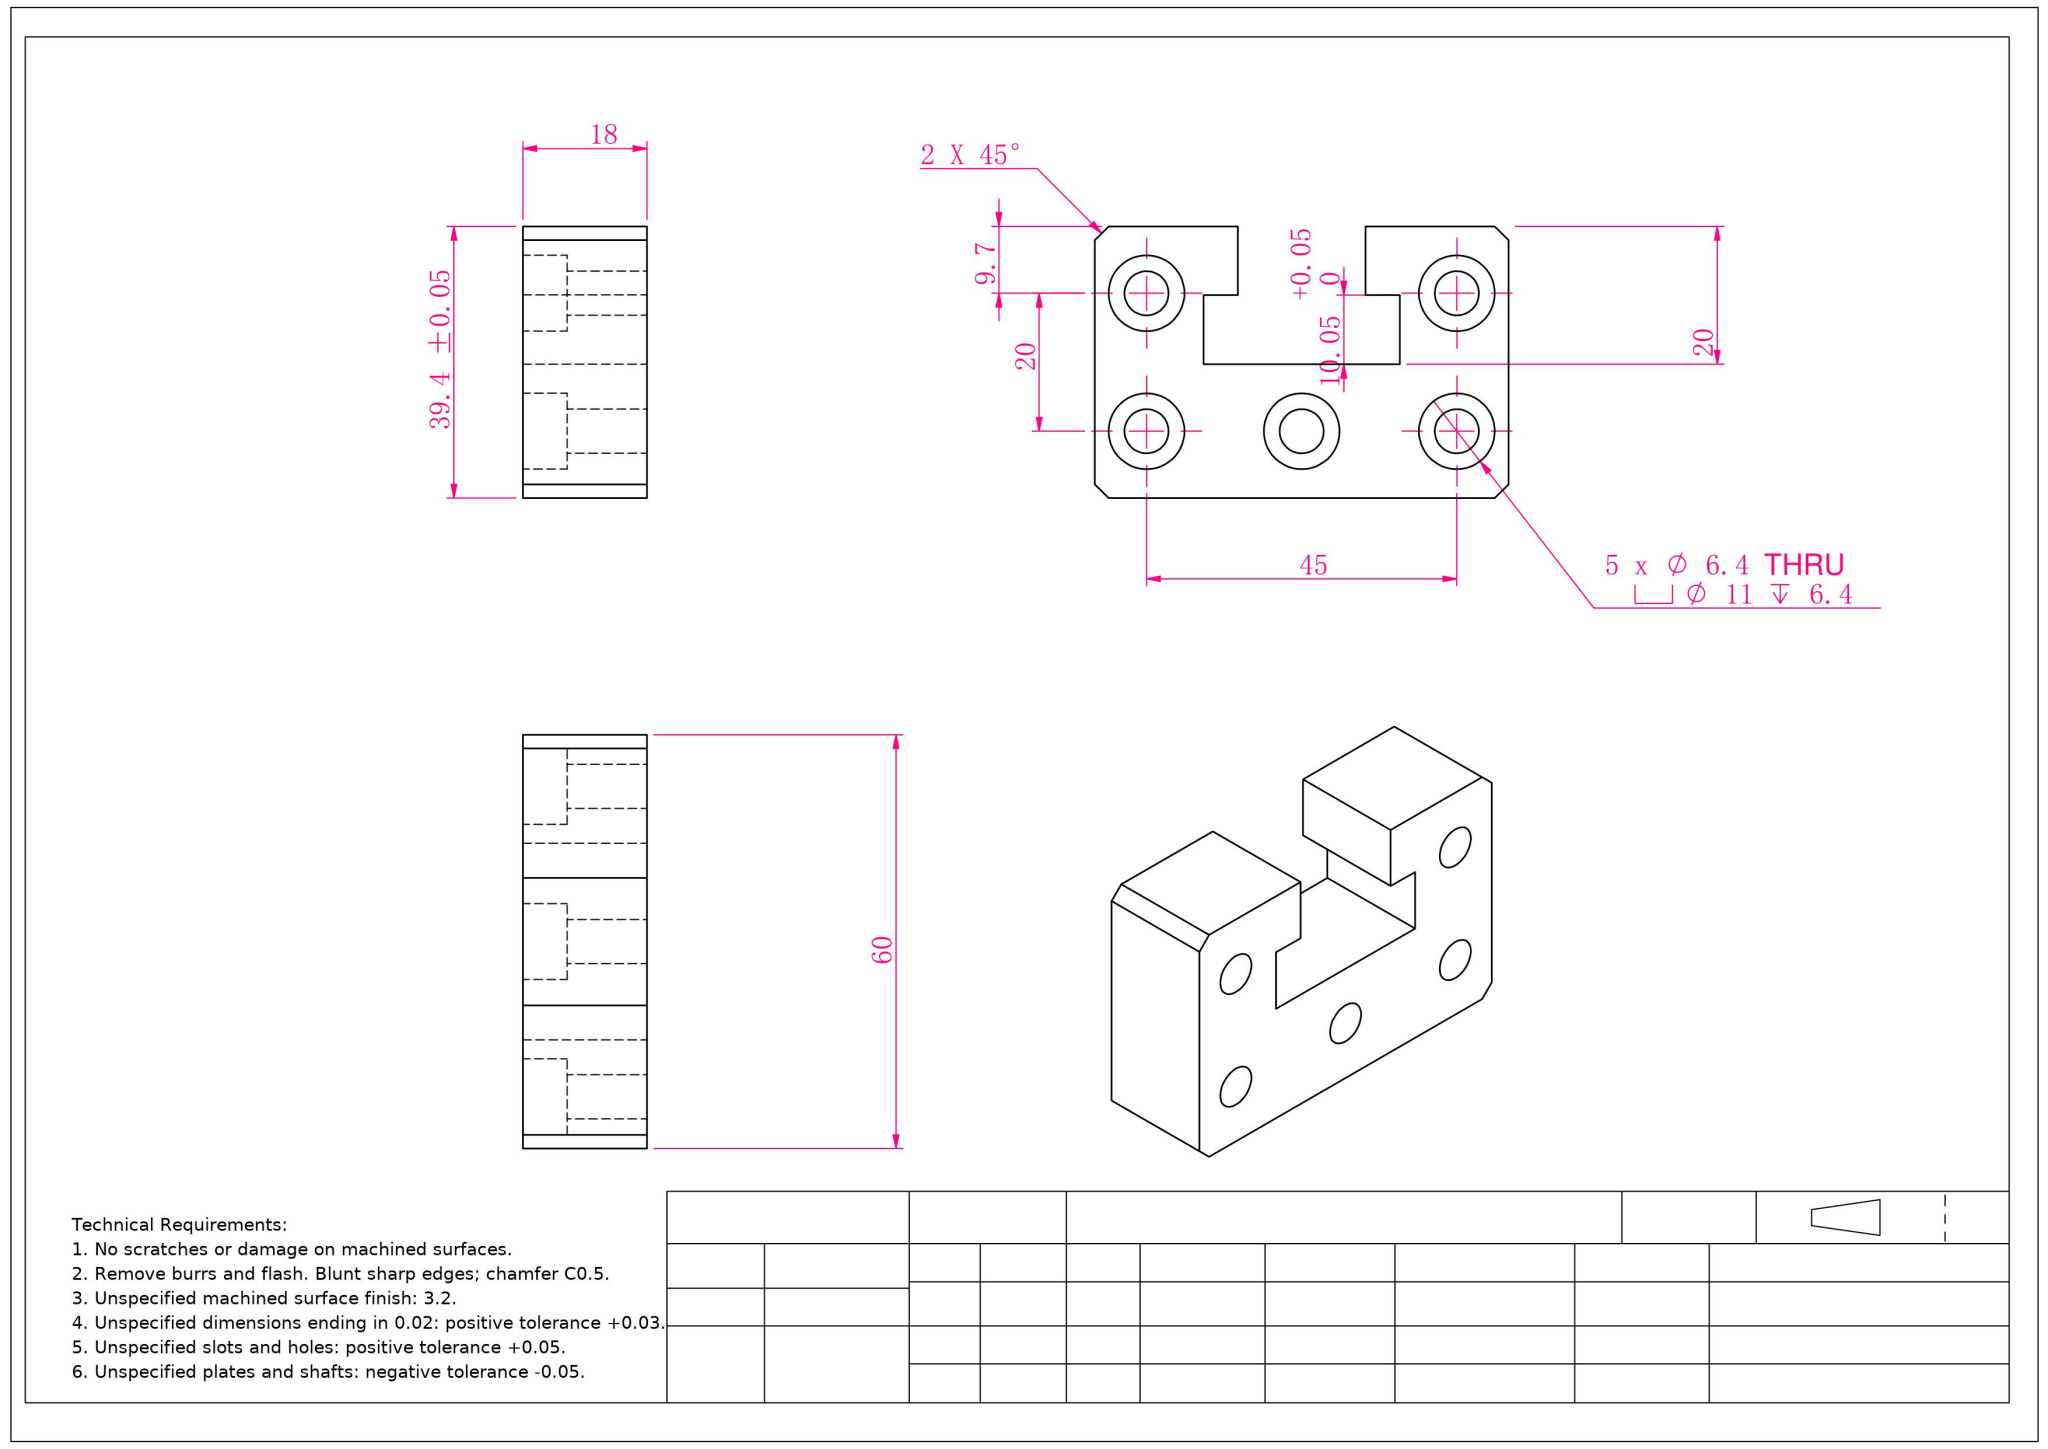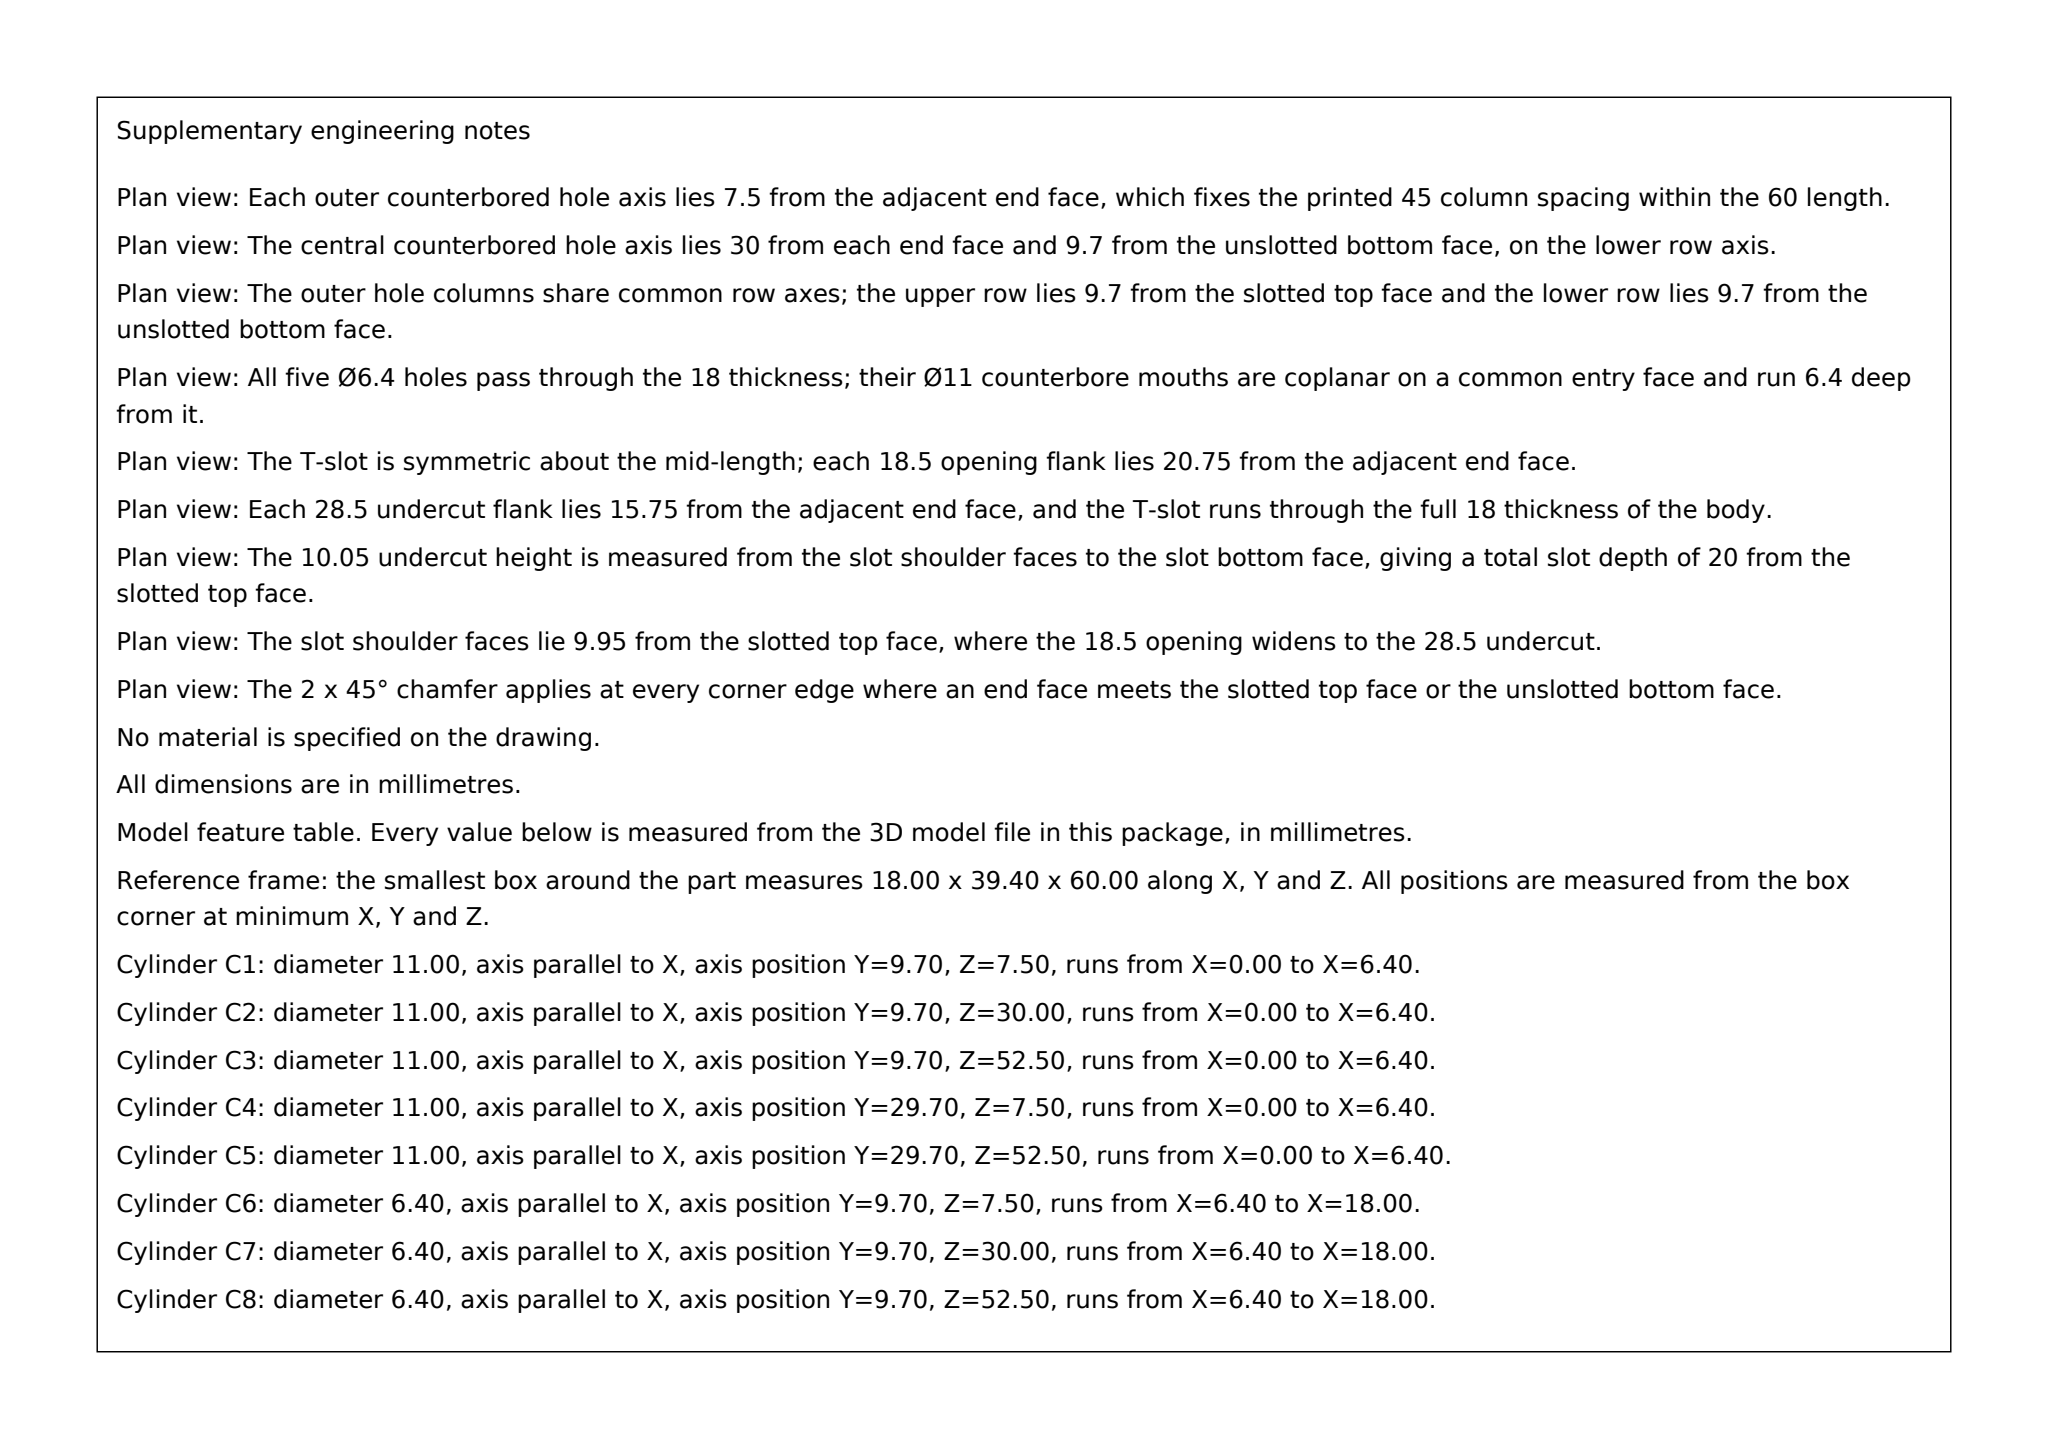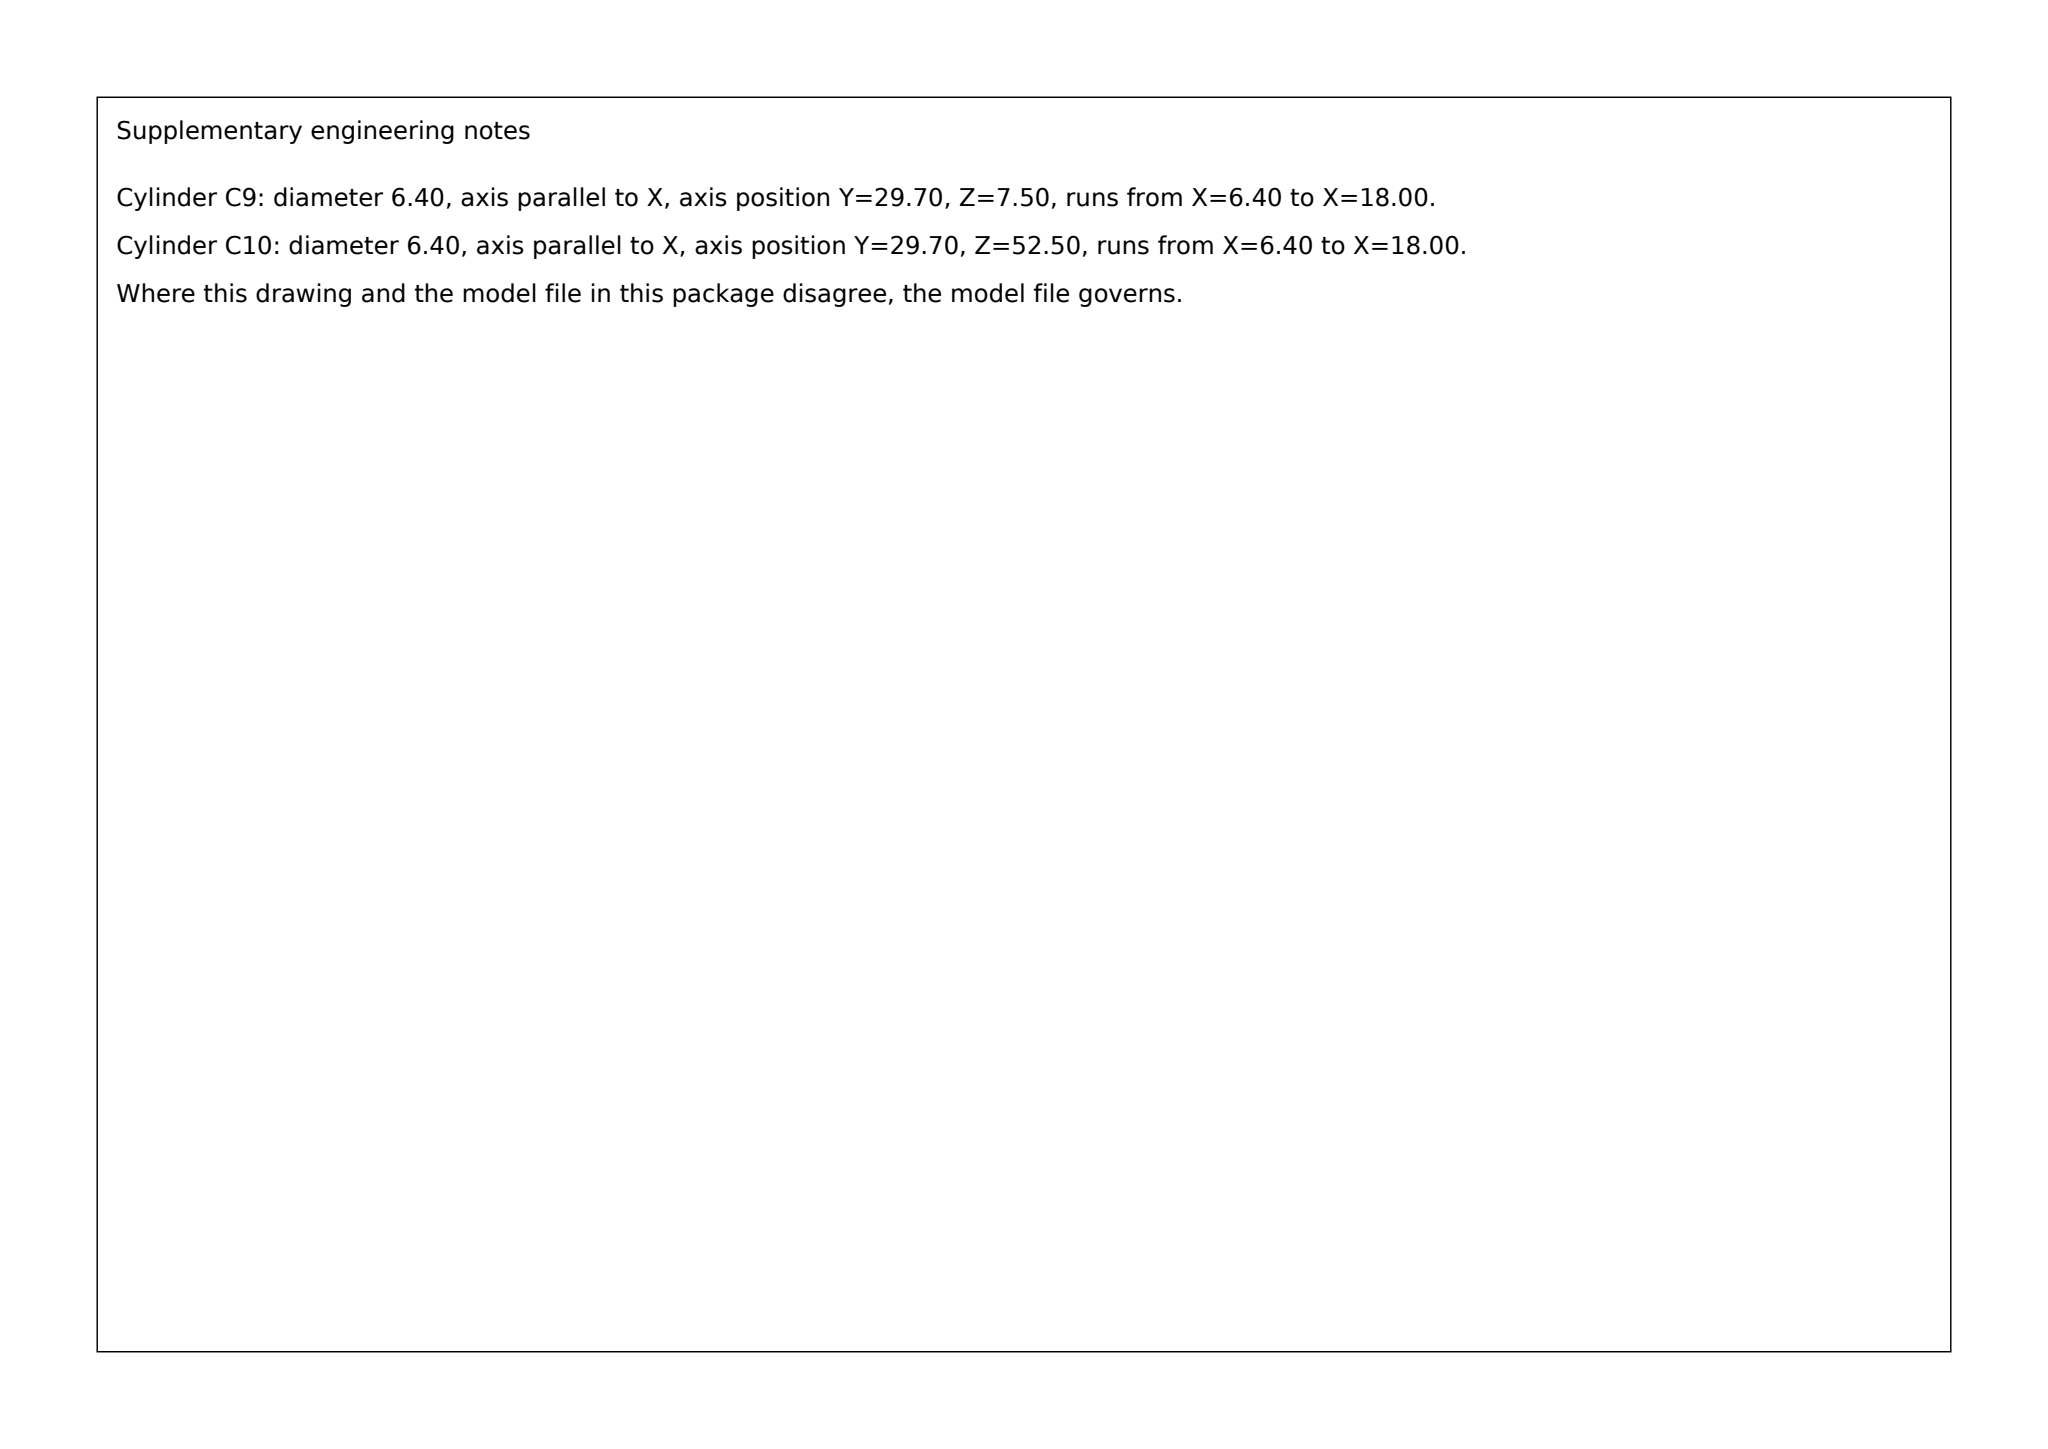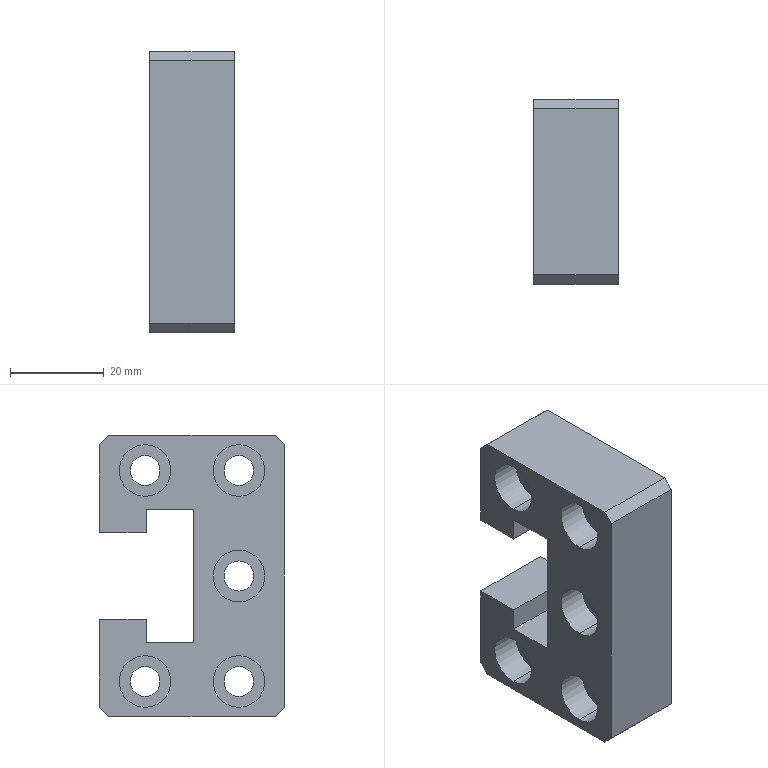Part | SolidWorks | mm | 1 solid | 43 faces | box 18 x 39.4 x 60 mm | volume 29032 mm3 | plane 23 | cylinder 20 | commonest cylinder face diameters 11 x10 6.4 x10
Drawing notes:
STEPPED SLOT: 18.5 WIDE DP 9.95; WIDENS TO 28.5 WIDE DP 20 FROM TOP | from the solid: z 20.75/39.25 = 18.5 wide; z 15.75/44.25 = 28.5 wide; y top 39.4, step floor y=29.45 (9.95 DP), slot floor y=19.4 (20 DP)
CHAMFER 2 X 45 TYP 4X CORNERS OF FRONT FACE (THRU 18 THK) | from the solid: Bbox 18x39.4x60; all four Y-Z face corners cut by 2x45 planes, full 18 depth along X
build123d program:
from build123d import *

# Parameters (mm, degrees)
SKETCH1_W                                       = 18
SKETCH1_H                                       = 39.4
BOSS_EXTRUDE1_DEPTH                             = 30
CUT_EXTRUDE1_DEPTH                              = 53.691
M6_HEX_SOCKET_HEAD_CAP_SCREW_CBORE1_D           = 6.4
M6_HEX_SOCKET_HEAD_CAP_SCREW_CBORE1_CBORE_D     = 11
M6_HEX_SOCKET_HEAD_CAP_SCREW_CBORE1_CBORE_DEPTH = 6.4
CHAMFER1_SIZE                                   = 2


with BuildPart() as part:
    # Sketch1 → Boss-Extrude1 (new, symmetric)
    with BuildSketch(Plane.XY):
        with Locations((0, 19.7)):
            Rectangle(SKETCH1_W, SKETCH1_H)
    extrude(amount=BOSS_EXTRUDE1_DEPTH, both=True)

    # Sketch2 → Cut-Extrude1 (cut, through all)
    with BuildSketch(Plane.ZY.offset(9)):
        Polygon((9.25, 29.45), (14.25, 29.45), (14.25, 19.4), (-14.25, 19.4), (-14.25, 29.45), (-9.25, 29.45), (-9.25, 39.4), (9.25, 39.4), align=None)
    extrude(amount=-CUT_EXTRUDE1_DEPTH, mode=Mode.SUBTRACT)

    # M6 Hex Socket Head Cap Screw CBORE1 (through all)
    with Locations(Plane.ZY.offset(9)):
        with Locations((-22.5, 29.7), (-22.5, 9.7), (22.5, 29.7), (22.5, 9.7), (0, 9.7)):
            CounterBoreHole(M6_HEX_SOCKET_HEAD_CAP_SCREW_CBORE1_D / 2, M6_HEX_SOCKET_HEAD_CAP_SCREW_CBORE1_CBORE_D / 2, M6_HEX_SOCKET_HEAD_CAP_SCREW_CBORE1_CBORE_DEPTH)

    # Chamfer1
    chamfer1_edges = [part.edges().sort_by_distance(p)[0] for p in [
        (0, 39.4, 30),
        (0, 39.4, -30),
        (0, 0, -30),
        (0, 0, 30),
    ]]
    chamfer(chamfer1_edges, length=CHAMFER1_SIZE)


solid = part.part